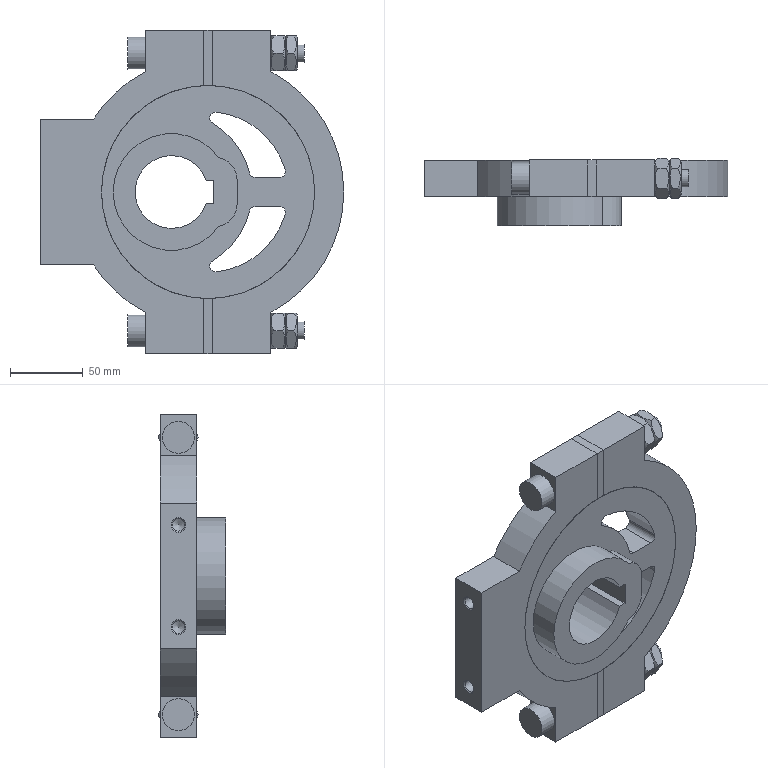Assembly | NX | mm | 11 component files | 13 solids | 172 faces | box 208 x 46.36 x 222 mm | volume 823631 mm3 | plane 108 | cylinder 52 | spline 8 | cone 4 | commonest cylinder face diameters 12 x14 152 x11 146 x6 8 x6 110 x4 186 x3 22 x2 32 x2
Bill of materials:
unnamed part 1 | 2 |  | Rectangular block-like plate with a single round through-hole and a shallow rectangular notch across one short edge, leaving two narrow raised tabs at the corners.
unnamed part 2 | 1 |  | Half-ring (semicircular saddle) with rectangular end lugs, each pierced by a small transverse hole, and a solid rectangular block on the outer side of the arc.
unnamed part 3 | 1 |  | Semicircular half-ring band with rectangular end lugs, each with a small transverse through-hole; no outer block.
unnamed part 4 | 1 |  | Flanged hub: circular flange disc with a smaller cylindrical boss on one side, a central bore with a single rectangular keyway, and two curved kidney-shaped through-slots in the flange.
unnamed part 5 | 2 |  | Hexagonal nut-shaped body with a central round through-bore and chamfered corners on both faces.
unnamed part 6 | 2 |  | Thin hexagonal nut-shaped body (jam-nut proportions) with a central round through-bore and chamfered corners on both faces.
unnamed part 7 | 2 |  | Headed cylindrical pin: a short larger-diameter cylindrical head with a long slender plain cylindrical shank and a flat end.
Mates:
1. fix | Strap_2 1 component
2. touch align | Strap_2 1 face | Sheave 1 face
3. touch align | Strap_2 1 face | Packing 2 face
4. touch align | Strap_2 1 face | Packing 2 face
5. touch align | Strap_2 1 face | Packing 2 face
6. touch align | Strap_2 1 face | Packing 1 face
7. touch align | Strap_2 1 face | Packing 1 face
8. touch align | Strap_2 1 face | Packing 1 face
9. touch align | Packing 2 face | Strap_1 1 face
10. touch align | Strap_1 1 face | Strap_2 1 face
11. touch align | Packing 1 face | Strap_1 1 face
12. touch align | Bolt_M12 2 face | Strap_2 1 face
13. touch align | Bolt_M12 2 face | Strap_2 1 face
14. touch align | Strap_2 1 face | Bolt_M12 2 face
15. touch align | Bolt_M12 2 face | Nut_M12 2 face
16. touch align | Strap_1 1 face | Nut_M12 2 face
17. touch align | Lock_Nut_M12 2 face | Bolt_M12 2 face
18. touch align | Lock_Nut_M12 2 face | Nut_M12 2 face